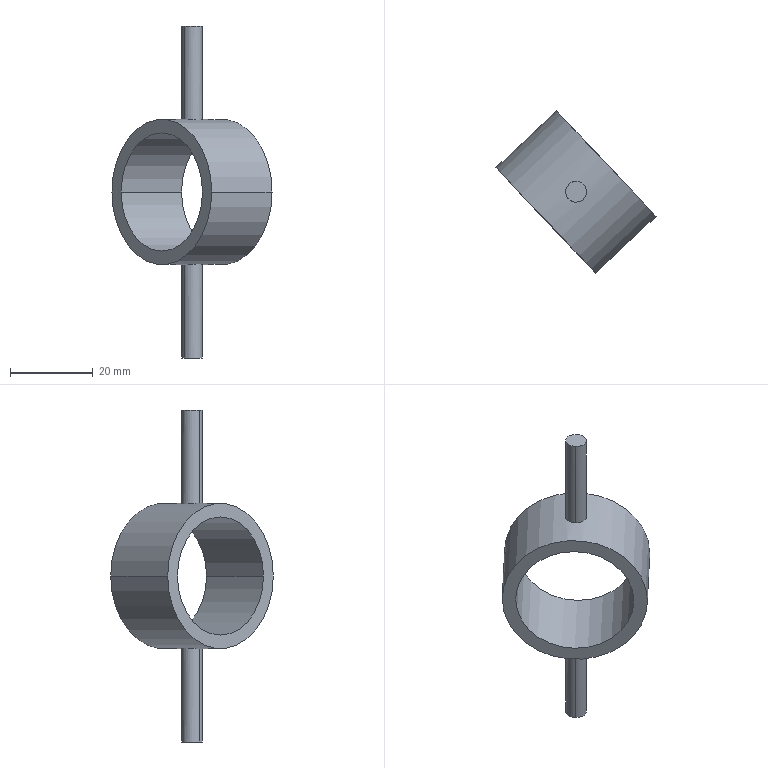Component | SolidWorks | ClampingMechanism-1_Sleeve-1 | 1 solid | 12 faces | box 38.57 x 39.18 x 80 mm | volume 7369 mm3 | cylinder 8 | plane 4 | commonest cylinder face diameters 5 x4 28.5 x2 35 x2
build123d program:
from build123d import *

# Parameters (mm, degrees)
SKETCH1_R           = 17.5
SKETCH1_R_2         = 14.25
BOSS_EXTRUDE1_DEPTH = 10
SKETCH2_R           = 2.5
BOSS_EXTRUDE2_DEPTH = 40
SKETCH3_R           = 14.25
CUT_EXTRUDE1_DEPTH  = 49.023


with BuildPart() as part:
    # Sketch1 → Boss-Extrude1 (new, symmetric)
    with BuildSketch(Plane.XY):
        Circle(SKETCH1_R)
        Circle(SKETCH1_R_2, mode=Mode.SUBTRACT)
    extrude(amount=BOSS_EXTRUDE1_DEPTH, both=True)

    # Sketch2 → Boss-Extrude2 (add, symmetric)
    with BuildSketch(Plane(origin=(0, 0, 0), x_dir=(1, 0, 0), z_dir=(0, 1, 0))):
        with Locations(Location((0, 0, 0), (0, 0, 90))):
            Circle(SKETCH2_R)
    extrude(amount=BOSS_EXTRUDE2_DEPTH, both=True)

    # Sketch3 → Cut-Extrude1 (cut, through all)
    with BuildSketch(Plane(origin=(0, 0, -10), x_dir=(-1, 0, 0), z_dir=(0, 0, -1))):
        with Locations(Location((0, 0, 0), (0, 0, 180))):
            Circle(SKETCH3_R)
    extrude(amount=-CUT_EXTRUDE1_DEPTH, mode=Mode.SUBTRACT)


solid = part.part

# Placed as in the assembly
solid = solid.moved(Location((-363.18, -233.51, -542.97), (90, -46.637, -180)))
STEP:
#1=COLOUR_RGB('',0.7922,0.8196,0.9333);
#2=FILL_AREA_STYLE_COLOUR('',#1);
#3=FILL_AREA_STYLE('',(#2));
#4=SURFACE_STYLE_FILL_AREA(#3);
#5=SURFACE_SIDE_STYLE('',(#4));
#6=SURFACE_STYLE_USAGE(.BOTH.,#5);
#7=PRESENTATION_STYLE_ASSIGNMENT((#6));
#8=CARTESIAN_POINT('',(-14.37,-9.261,-22.952));
#9=VERTEX_POINT('',#8);
#10=CARTESIAN_POINT('',(-14.227,-9.126,-22.952));
#11=VERTEX_POINT('',#10);
#12=CARTESIAN_POINT('',(-14.298,-9.193,-22.952));
#13=DIRECTION('',(-0.,0.,-1.));
#14=DIRECTION('',(-0.727,-0.6866,0.));
#15=AXIS2_PLACEMENT_3D('',#12,#13,#14);
#16=CIRCLE('',#15,0.09843);
#17=EDGE_CURVE('',#9,#11,#16,.T.);
#18=ORIENTED_EDGE('',*,*,#17,.F.);
#19=CARTESIAN_POINT('',(-14.37,-9.261,-22.066));
#20=VERTEX_POINT('',#19);
#21=CARTESIAN_POINT('',(-14.37,-9.261,-22.952));
#22=DIRECTION('',(0.,-0.,1.));
#23=VECTOR('',#22,39.37);
#24=LINE('',#21,#23);
#25=EDGE_CURVE('',#9,#20,#24,.T.);
#26=ORIENTED_EDGE('',*,*,#25,.T.);
#27=CARTESIAN_POINT('',(-14.227,-9.126,-22.066));
#28=VERTEX_POINT('',#27);
#29=CARTESIAN_POINT('',(-14.37,-9.261,-22.066));
#30=CARTESIAN_POINT('',(-14.374,-9.256,-22.066));
#31=CARTESIAN_POINT('',(-14.378,-9.251,-22.066));
#32=CARTESIAN_POINT('',(-14.385,-9.24,-22.065));
#33=CARTESIAN_POINT('',(-14.388,-9.234,-22.065));
#34=CARTESIAN_POINT('',(-14.393,-9.222,-22.064));
#35=CARTESIAN_POINT('',(-14.394,-9.216,-22.064));
#36=CARTESIAN_POINT('',(-14.397,-9.203,-22.063));
#37=CARTESIAN_POINT('',(-14.397,-9.197,-22.063));
#38=CARTESIAN_POINT('',(-14.397,-9.184,-22.062));
#39=CARTESIAN_POINT('',(-14.396,-9.178,-22.061));
#40=CARTESIAN_POINT('',(-14.393,-9.165,-22.06));
#41=CARTESIAN_POINT('',(-14.391,-9.159,-22.06));
#42=CARTESIAN_POINT('',(-14.386,-9.147,-22.059));
#43=CARTESIAN_POINT('',(-14.382,-9.142,-22.059));
#44=CARTESIAN_POINT('',(-14.375,-9.131,-22.059));
#45=CARTESIAN_POINT('',(-14.371,-9.126,-22.059));
#46=CARTESIAN_POINT('',(-14.361,-9.117,-22.059));
#47=CARTESIAN_POINT('',(-14.356,-9.113,-22.059));
#48=CARTESIAN_POINT('',(-14.345,-9.107,-22.059));
#49=CARTESIAN_POINT('',(-14.34,-9.104,-22.059));
#50=CARTESIAN_POINT('',(-14.327,-9.099,-22.06));
#51=CARTESIAN_POINT('',(-14.321,-9.097,-22.06));
#52=CARTESIAN_POINT('',(-14.309,-9.095,-22.061));
#53=CARTESIAN_POINT('',(-14.302,-9.095,-22.062));
#54=CARTESIAN_POINT('',(-14.283,-9.095,-22.063));
#55=CARTESIAN_POINT('',(-14.27,-9.098,-22.064));
#56=CARTESIAN_POINT('',(-14.252,-9.106,-22.065));
#57=CARTESIAN_POINT('',(-14.247,-9.109,-22.065));
#58=CARTESIAN_POINT('',(-14.236,-9.117,-22.066));
#59=CARTESIAN_POINT('',(-14.231,-9.121,-22.066));
#60=CARTESIAN_POINT('',(-14.227,-9.126,-22.066));
#61=B_SPLINE_CURVE_WITH_KNOTS('',3,(#29,#30,#31,#32,#33,#34,#35,#36,#37,#38,#39,#40,#41,#42,#43,#44,#45,#46,#47,#48,#49,#50,#51,#52,#53,#54,#55,#56,#57,#58,#59,#60),.UNSPECIFIED.,.F.,.F.,(4,2,2,2,2,2,2,2,2,2,2,2,2,2,2,4),(0.007826,0.008315,0.008804,0.009293,0.009782,0.01027,0.01076,0.01125,0.01174,0.01223,0.01272,0.01321,0.01369,0.01467,0.01516,0.01565),.UNSPECIFIED.);
#62=EDGE_CURVE('',#20,#28,#61,.T.);
#63=ORIENTED_EDGE('',*,*,#62,.T.);
#64=CARTESIAN_POINT('',(-14.227,-9.126,-22.952));
#65=DIRECTION('',(0.,-0.,1.));
#66=VECTOR('',#65,39.37);
#67=LINE('',#64,#66);
#68=EDGE_CURVE('',#11,#28,#67,.T.);
#69=ORIENTED_EDGE('',*,*,#68,.F.);
#70=EDGE_LOOP('',(#18,#26,#63,#69));
#71=FACE_OUTER_BOUND('',#70,.T.);
#72=CARTESIAN_POINT('',(-14.298,-9.193,-22.952));
#73=DIRECTION('',(0.,-0.,1.));
#74=DIRECTION('',(0.727,0.6866,0.));
#75=AXIS2_PLACEMENT_3D('',#72,#73,#74);
#76=CYLINDRICAL_SURFACE('',#75,0.09843);
#77=ADVANCED_FACE('',(#71),#76,.T.);
#78=CARTESIAN_POINT('',(-14.227,-9.126,-20.688));
#79=VERTEX_POINT('',#78);
#80=CARTESIAN_POINT('',(-14.37,-9.261,-20.688));
#81=VERTEX_POINT('',#80);
#82=CARTESIAN_POINT('',(-14.227,-9.126,-20.688));
#83=CARTESIAN_POINT('',(-14.231,-9.121,-20.688));
#84=CARTESIAN_POINT('',(-14.236,-9.117,-20.688));
#85=CARTESIAN_POINT('',(-14.247,-9.109,-20.688));
#86=CARTESIAN_POINT('',(-14.252,-9.106,-20.689));
#87=CARTESIAN_POINT('',(-14.264,-9.101,-20.689));
#88=CARTESIAN_POINT('',(-14.27,-9.099,-20.69));
#89=CARTESIAN_POINT('',(-14.283,-9.096,-20.69));
#90=CARTESIAN_POINT('',(-14.289,-9.095,-20.691));
#91=CARTESIAN_POINT('',(-14.302,-9.095,-20.692));
#92=CARTESIAN_POINT('',(-14.308,-9.095,-20.692));
#93=CARTESIAN_POINT('',(-14.321,-9.097,-20.693));
#94=CARTESIAN_POINT('',(-14.327,-9.099,-20.693));
#95=CARTESIAN_POINT('',(-14.339,-9.104,-20.694));
#96=CARTESIAN_POINT('',(-14.345,-9.106,-20.694));
#97=CARTESIAN_POINT('',(-14.356,-9.113,-20.695));
#98=CARTESIAN_POINT('',(-14.361,-9.117,-20.695));
#99=CARTESIAN_POINT('',(-14.371,-9.126,-20.695));
#100=CARTESIAN_POINT('',(-14.375,-9.131,-20.695));
#101=CARTESIAN_POINT('',(-14.382,-9.142,-20.694));
#102=CARTESIAN_POINT('',(-14.386,-9.147,-20.694));
#103=CARTESIAN_POINT('',(-14.391,-9.159,-20.693));
#104=CARTESIAN_POINT('',(-14.393,-9.165,-20.693));
#105=CARTESIAN_POINT('',(-14.396,-9.178,-20.692));
#106=CARTESIAN_POINT('',(-14.397,-9.184,-20.692));
#107=CARTESIAN_POINT('',(-14.397,-9.197,-20.691));
#108=CARTESIAN_POINT('',(-14.397,-9.203,-20.69));
#109=CARTESIAN_POINT('',(-14.394,-9.216,-20.69));
#110=CARTESIAN_POINT('',(-14.393,-9.222,-20.689));
#111=CARTESIAN_POINT('',(-14.388,-9.234,-20.688));
#112=CARTESIAN_POINT('',(-14.385,-9.24,-20.688));
#113=CARTESIAN_POINT('',(-14.378,-9.251,-20.688));
#114=CARTESIAN_POINT('',(-14.374,-9.256,-20.688));
#115=CARTESIAN_POINT('',(-14.37,-9.261,-20.688));
#116=B_SPLINE_CURVE_WITH_KNOTS('',3,(#82,#83,#84,#85,#86,#87,#88,#89,#90,#91,#92,#93,#94,#95,#96,#97,#98,#99,#100,#101,#102,#103,#104,#105,#106,#107,#108,#109,#110,#111,#112,#113,#114,#115),.UNSPECIFIED.,.F.,.F.,(4,2,2,2,2,2,2,2,2,2,2,2,2,2,2,2,4),(0.,0.0004891,0.0009783,0.001467,0.001957,0.002446,0.002935,0.003424,0.003913,0.004402,0.004891,0.00538,0.00587,0.006359,0.006848,0.007337,0.007826),.UNSPECIFIED.);
#117=EDGE_CURVE('',#79,#81,#116,.T.);
#118=ORIENTED_EDGE('',*,*,#117,.T.);
#119=CARTESIAN_POINT('',(-14.37,-9.261,-19.802));
#120=VERTEX_POINT('',#119);
#121=CARTESIAN_POINT('',(-14.37,-9.261,-22.952));
#122=DIRECTION('',(0.,-0.,1.));
#123=VECTOR('',#122,39.37);
#124=LINE('',#121,#123);
#125=EDGE_CURVE('',#81,#120,#124,.T.);
#126=ORIENTED_EDGE('',*,*,#125,.T.);
#127=CARTESIAN_POINT('',(-14.227,-9.126,-19.802));
#128=VERTEX_POINT('',#127);
#129=CARTESIAN_POINT('',(-14.298,-9.193,-19.802));
#130=DIRECTION('',(-0.,0.,-1.));
#131=DIRECTION('',(-0.727,-0.6866,0.));
#132=AXIS2_PLACEMENT_3D('',#129,#130,#131);
#133=CIRCLE('',#132,0.09843);
#134=EDGE_CURVE('',#120,#128,#133,.T.);
#135=ORIENTED_EDGE('',*,*,#134,.T.);
#136=CARTESIAN_POINT('',(-14.227,-9.126,-22.952));
#137=DIRECTION('',(0.,-0.,1.));
#138=VECTOR('',#137,39.37);
#139=LINE('',#136,#138);
#140=EDGE_CURVE('',#79,#128,#139,.T.);
#141=ORIENTED_EDGE('',*,*,#140,.F.);
#142=EDGE_LOOP('',(#118,#126,#135,#141));
#143=FACE_OUTER_BOUND('',#142,.T.);
#144=CARTESIAN_POINT('',(-14.298,-9.193,-22.952));
#145=DIRECTION('',(0.,-0.,1.));
#146=DIRECTION('',(0.727,0.6866,0.));
#147=AXIS2_PLACEMENT_3D('',#144,#145,#146);
#148=CYLINDRICAL_SURFACE('',#147,0.09843);
#149=ADVANCED_FACE('',(#143),#148,.T.);
#150=CARTESIAN_POINT('',(-14.199,-9.871,-21.377));
#151=VERTEX_POINT('',#150);
#152=CARTESIAN_POINT('',(-14.97,-9.056,-21.377));
#153=VERTEX_POINT('',#152);
#154=CARTESIAN_POINT('',(-14.585,-9.464,-21.377));
#155=DIRECTION('',(-0.727,-0.6866,-0.));
#156=DIRECTION('',(-0.6866,0.727,0.));
#157=AXIS2_PLACEMENT_3D('',#154,#155,#156);
#158=CIRCLE('',#157,0.561);
#159=EDGE_CURVE('',#151,#153,#158,.T.);
#160=ORIENTED_EDGE('',*,*,#159,.T.);
#161=CARTESIAN_POINT('',(-14.397,-8.515,-21.377));
#162=VERTEX_POINT('',#161);
#163=CARTESIAN_POINT('',(-14.97,-9.056,-21.377));
#164=DIRECTION('',(0.727,0.6866,0.));
#165=VECTOR('',#164,39.37);
#166=LINE('',#163,#165);
#167=EDGE_CURVE('',#153,#162,#166,.T.);
#168=ORIENTED_EDGE('',*,*,#167,.T.);
#169=CARTESIAN_POINT('',(-13.627,-9.331,-21.377));
#170=VERTEX_POINT('',#169);
#171=CARTESIAN_POINT('',(-14.012,-8.923,-21.377));
#172=DIRECTION('',(-0.727,-0.6866,-0.));
#173=DIRECTION('',(-0.6866,0.727,0.));
#174=AXIS2_PLACEMENT_3D('',#171,#172,#173);
#175=CIRCLE('',#174,0.561);
#176=EDGE_CURVE('',#170,#162,#175,.T.);
#177=ORIENTED_EDGE('',*,*,#176,.F.);
#178=CARTESIAN_POINT('',(-14.199,-9.871,-21.377));
#179=DIRECTION('',(0.727,0.6866,0.));
#180=VECTOR('',#179,39.37);
#181=LINE('',#178,#180);
#182=EDGE_CURVE('',#151,#170,#181,.T.);
#183=ORIENTED_EDGE('',*,*,#182,.F.);
#184=EDGE_LOOP('',(#160,#168,#177,#183));
#185=FACE_OUTER_BOUND('',#184,.T.);
#186=CARTESIAN_POINT('',(-14.585,-9.464,-21.377));
#187=DIRECTION('',(0.727,0.6866,0.));
#188=DIRECTION('',(0.6866,-0.727,0.));
#189=AXIS2_PLACEMENT_3D('',#186,#187,#188);
#190=CYLINDRICAL_SURFACE('',#189,0.561);
#191=ADVANCED_FACE('',(#185),#190,.F.);
#192=CARTESIAN_POINT('',(-14.227,-9.126,-22.066));
#193=CARTESIAN_POINT('',(-14.222,-9.13,-22.066));
#194=CARTESIAN_POINT('',(-14.218,-9.136,-22.066));
#195=CARTESIAN_POINT('',(-14.212,-9.146,-22.065));
#196=CARTESIAN_POINT('',(-14.209,-9.152,-22.065));
#197=CARTESIAN_POINT('',(-14.204,-9.164,-22.064));
#198=CARTESIAN_POINT('',(-14.202,-9.171,-22.064));
#199=CARTESIAN_POINT('',(-14.2,-9.183,-22.063));
#200=CARTESIAN_POINT('',(-14.2,-9.19,-22.063));
#201=CARTESIAN_POINT('',(-14.2,-9.203,-22.062));
#202=CARTESIAN_POINT('',(-14.201,-9.209,-22.061));
#203=CARTESIAN_POINT('',(-14.204,-9.222,-22.06));
#204=CARTESIAN_POINT('',(-14.206,-9.228,-22.06));
#205=CARTESIAN_POINT('',(-14.211,-9.239,-22.059));
#206=CARTESIAN_POINT('',(-14.214,-9.245,-22.059));
#207=CARTESIAN_POINT('',(-14.222,-9.256,-22.059));
#208=CARTESIAN_POINT('',(-14.226,-9.26,-22.059));
#209=CARTESIAN_POINT('',(-14.235,-9.269,-22.059));
#210=CARTESIAN_POINT('',(-14.241,-9.273,-22.059));
#211=CARTESIAN_POINT('',(-14.252,-9.28,-22.059));
#212=CARTESIAN_POINT('',(-14.257,-9.283,-22.059));
#213=CARTESIAN_POINT('',(-14.269,-9.288,-22.06));
#214=CARTESIAN_POINT('',(-14.276,-9.289,-22.06));
#215=CARTESIAN_POINT('',(-14.288,-9.291,-22.061));
#216=CARTESIAN_POINT('',(-14.295,-9.292,-22.062));
#217=CARTESIAN_POINT('',(-14.308,-9.292,-22.063));
#218=CARTESIAN_POINT('',(-14.314,-9.291,-22.063));
#219=CARTESIAN_POINT('',(-14.327,-9.288,-22.064));
#220=CARTESIAN_POINT('',(-14.333,-9.286,-22.064));
#221=CARTESIAN_POINT('',(-14.345,-9.28,-22.065));
#222=CARTESIAN_POINT('',(-14.35,-9.277,-22.065));
#223=CARTESIAN_POINT('',(-14.361,-9.27,-22.066));
#224=CARTESIAN_POINT('',(-14.366,-9.266,-22.066));
#225=CARTESIAN_POINT('',(-14.37,-9.261,-22.066));
#226=B_SPLINE_CURVE_WITH_KNOTS('',3,(#192,#193,#194,#195,#196,#197,#198,#199,#200,#201,#202,#203,#204,#205,#206,#207,#208,#209,#210,#211,#212,#213,#214,#215,#216,#217,#218,#219,#220,#221,#222,#223,#224,#225),.UNSPECIFIED.,.F.,.F.,(4,2,2,2,2,2,2,2,2,2,2,2,2,2,2,2,4),(0.,0.0004891,0.0009783,0.001467,0.001957,0.002446,0.002935,0.003424,0.003913,0.004402,0.004891,0.00538,0.00587,0.006359,0.006848,0.007337,0.007826),.UNSPECIFIED.);
#227=EDGE_CURVE('',#28,#20,#226,.T.);
#228=ORIENTED_EDGE('',*,*,#227,.F.);
#229=ORIENTED_EDGE('',*,*,#62,.F.);
#230=EDGE_LOOP('',(#228,#229));
#231=FACE_BOUND('',#230,.T.);
#232=CARTESIAN_POINT('',(-15.058,-8.963,-21.377));
#233=VERTEX_POINT('',#232);
#234=CARTESIAN_POINT('',(-14.112,-9.965,-21.377));
#235=VERTEX_POINT('',#234);
#236=CARTESIAN_POINT('',(-14.585,-9.464,-21.377));
#237=DIRECTION('',(-0.727,-0.6866,-0.));
#238=DIRECTION('',(-0.6866,0.727,0.));
#239=AXIS2_PLACEMENT_3D('',#236,#237,#238);
#240=CIRCLE('',#239,0.689);
#241=EDGE_CURVE('',#233,#235,#240,.T.);
#242=ORIENTED_EDGE('',*,*,#241,.F.);
#243=CARTESIAN_POINT('',(-14.485,-8.422,-21.377));
#244=VERTEX_POINT('',#243);
#245=CARTESIAN_POINT('',(-15.058,-8.963,-21.377));
#246=DIRECTION('',(0.727,0.6866,0.));
#247=VECTOR('',#246,39.37);
#248=LINE('',#245,#247);
#249=EDGE_CURVE('',#233,#244,#248,.T.);
#250=ORIENTED_EDGE('',*,*,#249,.T.);
#251=CARTESIAN_POINT('',(-13.539,-9.424,-21.377));
#252=VERTEX_POINT('',#251);
#253=CARTESIAN_POINT('',(-14.012,-8.923,-21.377));
#254=DIRECTION('',(-0.727,-0.6866,-0.));
#255=DIRECTION('',(-0.6866,0.727,0.));
#256=AXIS2_PLACEMENT_3D('',#253,#254,#255);
#257=CIRCLE('',#256,0.689);
#258=EDGE_CURVE('',#244,#252,#257,.T.);
#259=ORIENTED_EDGE('',*,*,#258,.T.);
#260=CARTESIAN_POINT('',(-14.112,-9.965,-21.377));
#261=DIRECTION('',(0.727,0.6866,0.));
#262=VECTOR('',#261,39.37);
#263=LINE('',#260,#262);
#264=EDGE_CURVE('',#235,#252,#263,.T.);
#265=ORIENTED_EDGE('',*,*,#264,.F.);
#266=EDGE_LOOP('',(#242,#250,#259,#265));
#267=FACE_OUTER_BOUND('',#266,.T.);
#268=CARTESIAN_POINT('',(-14.585,-9.464,-21.377));
#269=DIRECTION('',(0.727,0.6866,0.));
#270=DIRECTION('',(0.6866,-0.727,0.));
#271=AXIS2_PLACEMENT_3D('',#268,#269,#270);
#272=CYLINDRICAL_SURFACE('',#271,0.689);
#273=ADVANCED_FACE('',(#231,#267),#272,.T.);
#274=ORIENTED_EDGE('',*,*,#249,.F.);
#275=CARTESIAN_POINT('',(-14.585,-9.464,-21.377));
#276=DIRECTION('',(-0.727,-0.6866,-0.));
#277=DIRECTION('',(-0.6866,0.727,0.));
#278=AXIS2_PLACEMENT_3D('',#275,#276,#277);
#279=CIRCLE('',#278,0.689);
#280=EDGE_CURVE('',#235,#233,#279,.T.);
#281=ORIENTED_EDGE('',*,*,#280,.F.);
#282=ORIENTED_EDGE('',*,*,#264,.T.);
#283=CARTESIAN_POINT('',(-14.012,-8.923,-21.377));
#284=DIRECTION('',(-0.727,-0.6866,-0.));
#285=DIRECTION('',(-0.6866,0.727,0.));
#286=AXIS2_PLACEMENT_3D('',#283,#284,#285);
#287=CIRCLE('',#286,0.689);
#288=EDGE_CURVE('',#252,#244,#287,.T.);
#289=ORIENTED_EDGE('',*,*,#288,.T.);
#290=EDGE_LOOP('',(#274,#281,#282,#289));
#291=FACE_OUTER_BOUND('',#290,.T.);
#292=ORIENTED_EDGE('',*,*,#117,.F.);
#293=CARTESIAN_POINT('',(-14.37,-9.261,-20.688));
#294=CARTESIAN_POINT('',(-14.366,-9.266,-20.688));
#295=CARTESIAN_POINT('',(-14.361,-9.27,-20.688));
#296=CARTESIAN_POINT('',(-14.35,-9.277,-20.688));
#297=CARTESIAN_POINT('',(-14.345,-9.281,-20.688));
#298=CARTESIAN_POINT('',(-14.333,-9.286,-20.689));
#299=CARTESIAN_POINT('',(-14.327,-9.288,-20.69));
#300=CARTESIAN_POINT('',(-14.314,-9.291,-20.69));
#301=CARTESIAN_POINT('',(-14.308,-9.291,-20.691));
#302=CARTESIAN_POINT('',(-14.295,-9.292,-20.692));
#303=CARTESIAN_POINT('',(-14.288,-9.291,-20.692));
#304=CARTESIAN_POINT('',(-14.276,-9.289,-20.693));
#305=CARTESIAN_POINT('',(-14.27,-9.288,-20.693));
#306=CARTESIAN_POINT('',(-14.257,-9.283,-20.694));
#307=CARTESIAN_POINT('',(-14.252,-9.28,-20.694));
#308=CARTESIAN_POINT('',(-14.241,-9.273,-20.695));
#309=CARTESIAN_POINT('',(-14.236,-9.269,-20.695));
#310=CARTESIAN_POINT('',(-14.226,-9.26,-20.695));
#311=CARTESIAN_POINT('',(-14.222,-9.256,-20.695));
#312=CARTESIAN_POINT('',(-14.215,-9.245,-20.694));
#313=CARTESIAN_POINT('',(-14.211,-9.239,-20.694));
#314=CARTESIAN_POINT('',(-14.206,-9.228,-20.693));
#315=CARTESIAN_POINT('',(-14.204,-9.222,-20.693));
#316=CARTESIAN_POINT('',(-14.201,-9.209,-20.692));
#317=CARTESIAN_POINT('',(-14.2,-9.203,-20.692));
#318=CARTESIAN_POINT('',(-14.2,-9.183,-20.69));
#319=CARTESIAN_POINT('',(-14.202,-9.17,-20.689));
#320=CARTESIAN_POINT('',(-14.209,-9.152,-20.689));
#321=CARTESIAN_POINT('',(-14.212,-9.147,-20.688));
#322=CARTESIAN_POINT('',(-14.218,-9.136,-20.688));
#323=CARTESIAN_POINT('',(-14.222,-9.13,-20.688));
#324=CARTESIAN_POINT('',(-14.227,-9.126,-20.688));
#325=B_SPLINE_CURVE_WITH_KNOTS('',3,(#293,#294,#295,#296,#297,#298,#299,#300,#301,#302,#303,#304,#305,#306,#307,#308,#309,#310,#311,#312,#313,#314,#315,#316,#317,#318,#319,#320,#321,#322,#323,#324),.UNSPECIFIED.,.F.,.F.,(4,2,2,2,2,2,2,2,2,2,2,2,2,2,2,4),(0.007826,0.008315,0.008804,0.009293,0.009782,0.01027,0.01076,0.01125,0.01174,0.01223,0.01272,0.01321,0.01369,0.01467,0.01516,0.01565),.UNSPECIFIED.);
#326=EDGE_CURVE('',#81,#79,#325,.T.);
#327=ORIENTED_EDGE('',*,*,#326,.F.);
#328=EDGE_LOOP('',(#292,#327));
#329=FACE_BOUND('',#328,.T.);
#330=CARTESIAN_POINT('',(-14.585,-9.464,-21.377));
#331=DIRECTION('',(0.727,0.6866,0.));
#332=DIRECTION('',(0.6866,-0.727,0.));
#333=AXIS2_PLACEMENT_3D('',#330,#331,#332);
#334=CYLINDRICAL_SURFACE('',#333,0.689);
#335=ADVANCED_FACE('',(#291,#329),#334,.T.);
#336=ORIENTED_EDGE('',*,*,#167,.F.);
#337=CARTESIAN_POINT('',(-14.585,-9.464,-21.377));
#338=DIRECTION('',(-0.727,-0.6866,-0.));
#339=DIRECTION('',(-0.6866,0.727,0.));
#340=AXIS2_PLACEMENT_3D('',#337,#338,#339);
#341=CIRCLE('',#340,0.561);
#342=EDGE_CURVE('',#153,#151,#341,.T.);
#343=ORIENTED_EDGE('',*,*,#342,.T.);
#344=ORIENTED_EDGE('',*,*,#182,.T.);
#345=CARTESIAN_POINT('',(-14.012,-8.923,-21.377));
#346=DIRECTION('',(-0.727,-0.6866,-0.));
#347=DIRECTION('',(-0.6866,0.727,0.));
#348=AXIS2_PLACEMENT_3D('',#345,#346,#347);
#349=CIRCLE('',#348,0.561);
#350=EDGE_CURVE('',#162,#170,#349,.T.);
#351=ORIENTED_EDGE('',*,*,#350,.F.);
#352=EDGE_LOOP('',(#336,#343,#344,#351));
#353=FACE_OUTER_BOUND('',#352,.T.);
#354=CARTESIAN_POINT('',(-14.585,-9.464,-21.377));
#355=DIRECTION('',(0.727,0.6866,0.));
#356=DIRECTION('',(0.6866,-0.727,0.));
#357=AXIS2_PLACEMENT_3D('',#354,#355,#356);
#358=CYLINDRICAL_SURFACE('',#357,0.561);
#359=ADVANCED_FACE('',(#353),#358,.F.);
#360=ORIENTED_EDGE('',*,*,#280,.T.);
#361=ORIENTED_EDGE('',*,*,#241,.T.);
#362=EDGE_LOOP('',(#360,#361));
#363=FACE_OUTER_BOUND('',#362,.T.);
#364=ORIENTED_EDGE('',*,*,#159,.F.);
#365=ORIENTED_EDGE('',*,*,#342,.F.);
#366=EDGE_LOOP('',(#364,#365));
#367=FACE_BOUND('',#366,.T.);
#368=CARTESIAN_POINT('',(-14.585,-9.464,-21.377));
#369=DIRECTION('',(-0.727,-0.6866,-0.));
#370=DIRECTION('',(-0.6866,0.727,0.));
#371=AXIS2_PLACEMENT_3D('',#368,#369,#370);
#372=PLANE('',#371);
#373=ADVANCED_FACE('',(#363,#367),#372,.T.);
#374=ORIENTED_EDGE('',*,*,#288,.F.);
#375=ORIENTED_EDGE('',*,*,#258,.F.);
#376=EDGE_LOOP('',(#374,#375));
#377=FACE_OUTER_BOUND('',#376,.T.);
#378=ORIENTED_EDGE('',*,*,#176,.T.);
#379=ORIENTED_EDGE('',*,*,#350,.T.);
#380=EDGE_LOOP('',(#378,#379));
#381=FACE_BOUND('',#380,.T.);
#382=CARTESIAN_POINT('',(-14.012,-8.923,-21.377));
#383=DIRECTION('',(-0.727,-0.6866,-0.));
#384=DIRECTION('',(-0.6866,0.727,0.));
#385=AXIS2_PLACEMENT_3D('',#382,#383,#384);
#386=PLANE('',#385);
#387=ADVANCED_FACE('',(#377,#381),#386,.F.);
#388=CARTESIAN_POINT('',(-14.298,-9.193,-19.802));
#389=DIRECTION('',(-0.,0.,-1.));
#390=DIRECTION('',(-0.727,-0.6866,0.));
#391=AXIS2_PLACEMENT_3D('',#388,#389,#390);
#392=CIRCLE('',#391,0.09843);
#393=EDGE_CURVE('',#128,#120,#392,.T.);
#394=ORIENTED_EDGE('',*,*,#393,.F.);
#395=ORIENTED_EDGE('',*,*,#134,.F.);
#396=EDGE_LOOP('',(#394,#395));
#397=FACE_OUTER_BOUND('',#396,.T.);
#398=CARTESIAN_POINT('',(-14.298,-9.193,-19.802));
#399=DIRECTION('',(-0.,0.,-1.));
#400=DIRECTION('',(-0.727,-0.6866,-0.));
#401=AXIS2_PLACEMENT_3D('',#398,#399,#400);
#402=PLANE('',#401);
#403=ADVANCED_FACE('',(#397),#402,.F.);
#404=ORIENTED_EDGE('',*,*,#125,.F.);
#405=ORIENTED_EDGE('',*,*,#326,.T.);
#406=ORIENTED_EDGE('',*,*,#140,.T.);
#407=ORIENTED_EDGE('',*,*,#393,.T.);
#408=EDGE_LOOP('',(#404,#405,#406,#407));
#409=FACE_OUTER_BOUND('',#408,.T.);
#410=CARTESIAN_POINT('',(-14.298,-9.193,-22.952));
#411=DIRECTION('',(0.,-0.,1.));
#412=DIRECTION('',(0.727,0.6866,0.));
#413=AXIS2_PLACEMENT_3D('',#410,#411,#412);
#414=CYLINDRICAL_SURFACE('',#413,0.09843);
#415=ADVANCED_FACE('',(#409),#414,.T.);
#416=ORIENTED_EDGE('',*,*,#25,.F.);
#417=CARTESIAN_POINT('',(-14.298,-9.193,-22.952));
#418=DIRECTION('',(-0.,0.,-1.));
#419=DIRECTION('',(-0.727,-0.6866,0.));
#420=AXIS2_PLACEMENT_3D('',#417,#418,#419);
#421=CIRCLE('',#420,0.09843);
#422=EDGE_CURVE('',#11,#9,#421,.T.);
#423=ORIENTED_EDGE('',*,*,#422,.F.);
#424=ORIENTED_EDGE('',*,*,#68,.T.);
#425=ORIENTED_EDGE('',*,*,#227,.T.);
#426=EDGE_LOOP('',(#416,#423,#424,#425));
#427=FACE_OUTER_BOUND('',#426,.T.);
#428=CARTESIAN_POINT('',(-14.298,-9.193,-22.952));
#429=DIRECTION('',(0.,-0.,1.));
#430=DIRECTION('',(0.727,0.6866,0.));
#431=AXIS2_PLACEMENT_3D('',#428,#429,#430);
#432=CYLINDRICAL_SURFACE('',#431,0.09843);
#433=ADVANCED_FACE('',(#427),#432,.T.);
#434=ORIENTED_EDGE('',*,*,#422,.T.);
#435=ORIENTED_EDGE('',*,*,#17,.T.);
#436=EDGE_LOOP('',(#434,#435));
#437=FACE_OUTER_BOUND('',#436,.T.);
#438=CARTESIAN_POINT('',(-14.298,-9.193,-22.952));
#439=DIRECTION('',(-0.,0.,-1.));
#440=DIRECTION('',(-0.727,-0.6866,-0.));
#441=AXIS2_PLACEMENT_3D('',#438,#439,#440);
#442=PLANE('',#441);
#443=ADVANCED_FACE('',(#437),#442,.T.);
#444=CLOSED_SHELL('',(#77,#149,#191,#273,#335,#359,#373,#387,#403,#415,#433,#443));
#445=MANIFOLD_SOLID_BREP('',#444);
#446=STYLED_ITEM('',(#7),#445);
#447=PRESENTATION_LAYER_ASSIGNMENT('','',(#446));
#448=(LENGTH_UNIT()NAMED_UNIT(*)SI_UNIT($,.METRE.));
#449=LENGTH_MEASURE_WITH_UNIT(LENGTH_MEASURE(0.0254),#448);
#450=DIMENSIONAL_EXPONENTS(1.,0.,0.,0.,0.,0.,0.);
#451=(CONVERSION_BASED_UNIT('',#449)LENGTH_UNIT()NAMED_UNIT(#450));
#452=UNCERTAINTY_MEASURE_WITH_UNIT(LENGTH_MEASURE(0.00001),#451,'','');
#453=(NAMED_UNIT(*)PLANE_ANGLE_UNIT()SI_UNIT($,.RADIAN.));
#454=(NAMED_UNIT(*)SI_UNIT($,.STERADIAN.)SOLID_ANGLE_UNIT());
#455=(GEOMETRIC_REPRESENTATION_CONTEXT(3)GLOBAL_UNCERTAINTY_ASSIGNED_CONTEXT((#452))GLOBAL_UNIT_ASSIGNED_CONTEXT((#451,#453,#454))REPRESENTATION_CONTEXT('',''));
#456=MECHANICAL_DESIGN_GEOMETRIC_PRESENTATION_REPRESENTATION('',(#446),#455);
#457=CARTESIAN_POINT('',(0.,0.,0.));
#458=DIRECTION('',(0.,0.,1.));
#459=DIRECTION('',(1.,0.,0.));
#460=AXIS2_PLACEMENT_3D('',#457,#458,#459);
#461=(LENGTH_UNIT()NAMED_UNIT(*)SI_UNIT($,.METRE.));
#462=LENGTH_MEASURE_WITH_UNIT(LENGTH_MEASURE(0.0254),#461);
#463=DIMENSIONAL_EXPONENTS(1.,0.,0.,0.,0.,0.,0.);
#464=(CONVERSION_BASED_UNIT('',#462)LENGTH_UNIT()NAMED_UNIT(#463));
#465=UNCERTAINTY_MEASURE_WITH_UNIT(LENGTH_MEASURE(0.00001),#464,'','');
#466=(NAMED_UNIT(*)PLANE_ANGLE_UNIT()SI_UNIT($,.RADIAN.));
#467=(NAMED_UNIT(*)SI_UNIT($,.STERADIAN.)SOLID_ANGLE_UNIT());
#468=(GEOMETRIC_REPRESENTATION_CONTEXT(3)GLOBAL_UNCERTAINTY_ASSIGNED_CONTEXT((#465))GLOBAL_UNIT_ASSIGNED_CONTEXT((#464,#466,#467))REPRESENTATION_CONTEXT('',''));
#469=ADVANCED_BREP_SHAPE_REPRESENTATION('',(#445,#460),#468);